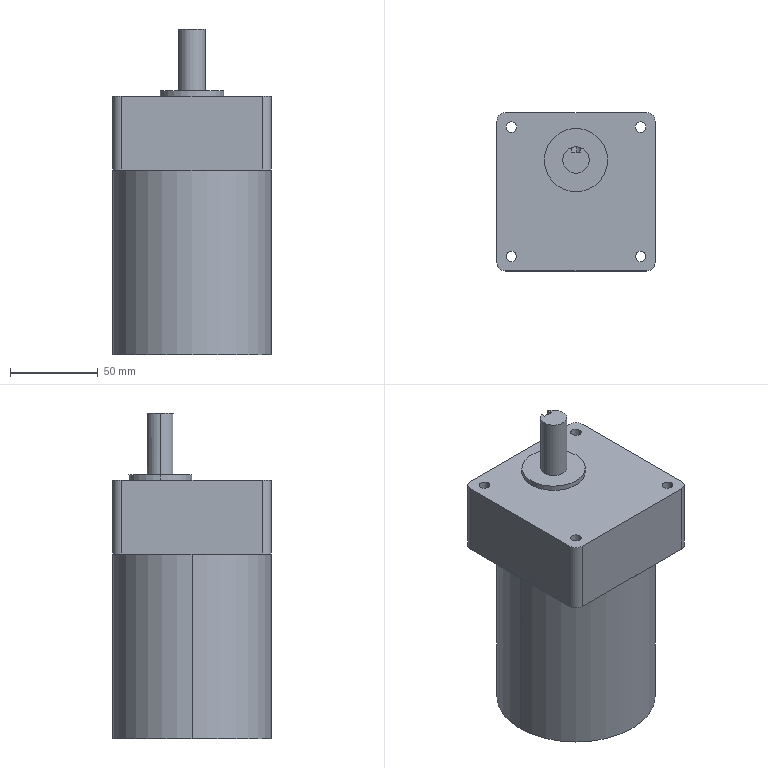Component | SolidWorks | YN90G60 90JA40G15-1 | 1 solid | 35 faces | box 90 x 90 x 185 mm | volume 1011347 mm3 | cylinder 20 | plane 15 | commonest cylinder face diameters 6 x8 10 x4 90 x2 15 x2 36 x2 5 x2
STEP:
#1=CARTESIAN_POINT('',(-1.772,4.705,-1.457));
#2=VERTEX_POINT('',#1);
#3=CARTESIAN_POINT('',(1.772,4.705,-1.457));
#4=VERTEX_POINT('',#3);
#5=CARTESIAN_POINT('',(0.,4.705,-1.457));
#6=DIRECTION('',(0.,0.,-1.));
#7=DIRECTION('',(-1.,0.,0.));
#8=AXIS2_PLACEMENT_3D('',#5,#6,#7);
#9=CIRCLE('',#8,1.772);
#10=EDGE_CURVE('',#2,#4,#9,.T.);
#11=ORIENTED_EDGE('',*,*,#10,.F.);
#12=CARTESIAN_POINT('',(-1.772,4.705,2.677));
#13=VERTEX_POINT('',#12);
#14=CARTESIAN_POINT('',(-1.772,4.705,-1.457));
#15=DIRECTION('',(0.,0.,1.));
#16=VECTOR('',#15,39.37);
#17=LINE('',#14,#16);
#18=EDGE_CURVE('',#2,#13,#17,.T.);
#19=ORIENTED_EDGE('',*,*,#18,.T.);
#20=CARTESIAN_POINT('',(0.,6.476,2.677));
#21=VERTEX_POINT('',#20);
#22=CARTESIAN_POINT('',(0.,4.705,2.677));
#23=DIRECTION('',(0.,0.,-1.));
#24=DIRECTION('',(-1.,0.,0.));
#25=AXIS2_PLACEMENT_3D('',#22,#23,#24);
#26=CIRCLE('',#25,1.772);
#27=EDGE_CURVE('',#13,#21,#26,.T.);
#28=ORIENTED_EDGE('',*,*,#27,.T.);
#29=CARTESIAN_POINT('',(1.772,4.705,2.677));
#30=VERTEX_POINT('',#29);
#31=CARTESIAN_POINT('',(0.,4.705,2.677));
#32=DIRECTION('',(0.,0.,-1.));
#33=DIRECTION('',(-1.,0.,0.));
#34=AXIS2_PLACEMENT_3D('',#31,#32,#33);
#35=CIRCLE('',#34,1.772);
#36=EDGE_CURVE('',#21,#30,#35,.T.);
#37=ORIENTED_EDGE('',*,*,#36,.T.);
#38=CARTESIAN_POINT('',(1.772,4.705,-1.457));
#39=DIRECTION('',(0.,0.,1.));
#40=VECTOR('',#39,39.37);
#41=LINE('',#38,#40);
#42=EDGE_CURVE('',#4,#30,#41,.T.);
#43=ORIENTED_EDGE('',*,*,#42,.F.);
#44=EDGE_LOOP('',(#11,#19,#28,#37,#43));
#45=FACE_OUTER_BOUND('',#44,.T.);
#46=CARTESIAN_POINT('',(0.,4.705,-1.457));
#47=DIRECTION('',(0.,0.,1.));
#48=DIRECTION('',(1.,0.,0.));
#49=AXIS2_PLACEMENT_3D('',#46,#47,#48);
#50=CYLINDRICAL_SURFACE('',#49,1.772);
#51=ADVANCED_FACE('',(#45),#50,.T.);
#52=CARTESIAN_POINT('',(0.2953,5.413,5.827));
#53=VERTEX_POINT('',#52);
#54=CARTESIAN_POINT('',(0.09843,5.692,5.827));
#55=VERTEX_POINT('',#54);
#56=CARTESIAN_POINT('',(0.,5.413,5.827));
#57=DIRECTION('',(0.,0.,1.));
#58=DIRECTION('',(1.,0.,0.));
#59=AXIS2_PLACEMENT_3D('',#56,#57,#58);
#60=CIRCLE('',#59,0.2953);
#61=EDGE_CURVE('',#53,#55,#60,.T.);
#62=ORIENTED_EDGE('',*,*,#61,.F.);
#63=CARTESIAN_POINT('',(0.2953,5.413,4.449));
#64=VERTEX_POINT('',#63);
#65=CARTESIAN_POINT('',(0.2953,5.413,5.827));
#66=DIRECTION('',(0.,0.,-1.));
#67=VECTOR('',#66,39.37);
#68=LINE('',#65,#67);
#69=EDGE_CURVE('',#53,#64,#68,.T.);
#70=ORIENTED_EDGE('',*,*,#69,.T.);
#71=CARTESIAN_POINT('',(-0.2953,5.413,4.449));
#72=VERTEX_POINT('',#71);
#73=CARTESIAN_POINT('',(0.,5.413,4.449));
#74=DIRECTION('',(0.,0.,1.));
#75=DIRECTION('',(1.,0.,0.));
#76=AXIS2_PLACEMENT_3D('',#73,#74,#75);
#77=CIRCLE('',#76,0.2953);
#78=EDGE_CURVE('',#64,#72,#77,.T.);
#79=ORIENTED_EDGE('',*,*,#78,.T.);
#80=CARTESIAN_POINT('',(-0.2953,5.413,5.827));
#81=VERTEX_POINT('',#80);
#82=CARTESIAN_POINT('',(-0.2953,5.413,5.827));
#83=DIRECTION('',(0.,0.,-1.));
#84=VECTOR('',#83,39.37);
#85=LINE('',#82,#84);
#86=EDGE_CURVE('',#81,#72,#85,.T.);
#87=ORIENTED_EDGE('',*,*,#86,.F.);
#88=CARTESIAN_POINT('',(-0.09843,5.692,5.827));
#89=VERTEX_POINT('',#88);
#90=CARTESIAN_POINT('',(0.,5.413,5.827));
#91=DIRECTION('',(0.,0.,1.));
#92=DIRECTION('',(1.,0.,0.));
#93=AXIS2_PLACEMENT_3D('',#90,#91,#92);
#94=CIRCLE('',#93,0.2953);
#95=EDGE_CURVE('',#89,#81,#94,.T.);
#96=ORIENTED_EDGE('',*,*,#95,.F.);
#97=CARTESIAN_POINT('',(-0.09843,5.692,4.744));
#98=VERTEX_POINT('',#97);
#99=CARTESIAN_POINT('',(-0.09843,5.692,5.827));
#100=DIRECTION('',(0.,0.,-1.));
#101=VECTOR('',#100,39.37);
#102=LINE('',#99,#101);
#103=EDGE_CURVE('',#89,#98,#102,.T.);
#104=ORIENTED_EDGE('',*,*,#103,.T.);
#105=CARTESIAN_POINT('',(0.,5.709,4.646));
#106=VERTEX_POINT('',#105);
#107=CARTESIAN_POINT('',(-0.09843,5.692,4.744));
#108=CARTESIAN_POINT('',(-0.09843,5.692,4.738));
#109=CARTESIAN_POINT('',(-0.09778,5.692,4.731));
#110=CARTESIAN_POINT('',(-0.09525,5.693,4.718));
#111=CARTESIAN_POINT('',(-0.09334,5.694,4.712));
#112=CARTESIAN_POINT('',(-0.08839,5.695,4.7));
#113=CARTESIAN_POINT('',(-0.08537,5.696,4.695));
#114=CARTESIAN_POINT('',(-0.07824,5.698,4.684));
#115=CARTESIAN_POINT('',(-0.07412,5.699,4.679));
#116=CARTESIAN_POINT('',(-0.06062,5.703,4.666));
#117=CARTESIAN_POINT('',(-0.04973,5.705,4.658));
#118=CARTESIAN_POINT('',(-0.032,5.707,4.651));
#119=CARTESIAN_POINT('',(-0.02576,5.708,4.649));
#120=CARTESIAN_POINT('',(-0.01301,5.708,4.646));
#121=CARTESIAN_POINT('',(-0.006549,5.709,4.646));
#122=CARTESIAN_POINT('',(0.,5.709,4.646));
#123=B_SPLINE_CURVE_WITH_KNOTS('',3,(#107,#108,#109,#110,#111,#112,#113,#114,#115,#116,#117,#118,#119,#120,#121,#122),.UNSPECIFIED.,.F.,.F.,(4,2,2,2,2,2,2,4),(0.,0.0004917,0.0009834,0.001475,0.001967,0.00295,0.003442,0.003934),.UNSPECIFIED.);
#124=EDGE_CURVE('',#98,#106,#123,.T.);
#125=ORIENTED_EDGE('',*,*,#124,.T.);
#126=CARTESIAN_POINT('',(0.09843,5.692,4.744));
#127=VERTEX_POINT('',#126);
#128=CARTESIAN_POINT('',(0.,5.709,4.646));
#129=CARTESIAN_POINT('',(0.00655,5.709,4.646));
#130=CARTESIAN_POINT('',(0.01298,5.708,4.646));
#131=CARTESIAN_POINT('',(0.02562,5.708,4.649));
#132=CARTESIAN_POINT('',(0.03189,5.707,4.651));
#133=CARTESIAN_POINT('',(0.04379,5.705,4.656));
#134=CARTESIAN_POINT('',(0.04942,5.705,4.659));
#135=CARTESIAN_POINT('',(0.06008,5.703,4.666));
#136=CARTESIAN_POINT('',(0.06509,5.701,4.67));
#137=CARTESIAN_POINT('',(0.0786,5.698,4.683));
#138=CARTESIAN_POINT('',(0.08591,5.696,4.694));
#139=CARTESIAN_POINT('',(0.0933,5.694,4.712));
#140=CARTESIAN_POINT('',(0.09522,5.693,4.718));
#141=CARTESIAN_POINT('',(0.09778,5.692,4.731));
#142=CARTESIAN_POINT('',(0.09843,5.692,4.738));
#143=CARTESIAN_POINT('',(0.09843,5.692,4.744));
#144=B_SPLINE_CURVE_WITH_KNOTS('',3,(#128,#129,#130,#131,#132,#133,#134,#135,#136,#137,#138,#139,#140,#141,#142,#143),.UNSPECIFIED.,.F.,.F.,(4,2,2,2,2,2,2,4),(0.,0.0004917,0.0009835,0.001475,0.001967,0.00295,0.003442,0.003934),.UNSPECIFIED.);
#145=EDGE_CURVE('',#106,#127,#144,.T.);
#146=ORIENTED_EDGE('',*,*,#145,.T.);
#147=CARTESIAN_POINT('',(0.09843,5.692,5.827));
#148=DIRECTION('',(0.,0.,1.));
#149=VECTOR('',#148,39.37);
#150=LINE('',#147,#149);
#151=EDGE_CURVE('',#127,#55,#150,.T.);
#152=ORIENTED_EDGE('',*,*,#151,.T.);
#153=EDGE_LOOP('',(#62,#70,#79,#87,#96,#104,#125,#146,#152));
#154=FACE_OUTER_BOUND('',#153,.T.);
#155=CARTESIAN_POINT('',(0.,5.413,5.827));
#156=DIRECTION('',(0.,0.,-1.));
#157=DIRECTION('',(-1.,0.,0.));
#158=AXIS2_PLACEMENT_3D('',#155,#156,#157);
#159=CYLINDRICAL_SURFACE('',#158,0.2953);
#160=ADVANCED_FACE('',(#154),#159,.T.);
#161=CARTESIAN_POINT('',(0.7087,5.413,4.449));
#162=VERTEX_POINT('',#161);
#163=CARTESIAN_POINT('',(-0.7087,5.413,4.449));
#164=VERTEX_POINT('',#163);
#165=CARTESIAN_POINT('',(0.,5.413,4.449));
#166=DIRECTION('',(0.,0.,1.));
#167=DIRECTION('',(1.,0.,0.));
#168=AXIS2_PLACEMENT_3D('',#165,#166,#167);
#169=CIRCLE('',#168,0.7087);
#170=EDGE_CURVE('',#162,#164,#169,.T.);
#171=ORIENTED_EDGE('',*,*,#170,.F.);
#172=CARTESIAN_POINT('',(0.7087,5.413,4.331));
#173=VERTEX_POINT('',#172);
#174=CARTESIAN_POINT('',(0.7087,5.413,4.449));
#175=DIRECTION('',(0.,0.,-1.));
#176=VECTOR('',#175,39.37);
#177=LINE('',#174,#176);
#178=EDGE_CURVE('',#162,#173,#177,.T.);
#179=ORIENTED_EDGE('',*,*,#178,.T.);
#180=CARTESIAN_POINT('',(-0.7087,5.413,4.331));
#181=VERTEX_POINT('',#180);
#182=CARTESIAN_POINT('',(0.,5.413,4.331));
#183=DIRECTION('',(0.,0.,1.));
#184=DIRECTION('',(1.,0.,0.));
#185=AXIS2_PLACEMENT_3D('',#182,#183,#184);
#186=CIRCLE('',#185,0.7087);
#187=EDGE_CURVE('',#173,#181,#186,.T.);
#188=ORIENTED_EDGE('',*,*,#187,.T.);
#189=CARTESIAN_POINT('',(-0.7087,5.413,4.449));
#190=DIRECTION('',(0.,0.,-1.));
#191=VECTOR('',#190,39.37);
#192=LINE('',#189,#191);
#193=EDGE_CURVE('',#164,#181,#192,.T.);
#194=ORIENTED_EDGE('',*,*,#193,.F.);
#195=EDGE_LOOP('',(#171,#179,#188,#194));
#196=FACE_OUTER_BOUND('',#195,.T.);
#197=CARTESIAN_POINT('',(0.,5.413,4.449));
#198=DIRECTION('',(0.,0.,-1.));
#199=DIRECTION('',(-1.,0.,0.));
#200=AXIS2_PLACEMENT_3D('',#197,#198,#199);
#201=CYLINDRICAL_SURFACE('',#200,0.7087);
#202=ADVANCED_FACE('',(#196),#201,.T.);
#203=CARTESIAN_POINT('',(1.33,3.257,4.331));
#204=VERTEX_POINT('',#203);
#205=CARTESIAN_POINT('',(1.566,3.257,4.331));
#206=VERTEX_POINT('',#205);
#207=CARTESIAN_POINT('',(1.448,3.257,4.331));
#208=DIRECTION('',(0.,0.,1.));
#209=DIRECTION('',(1.,0.,0.));
#210=AXIS2_PLACEMENT_3D('',#207,#208,#209);
#211=CIRCLE('',#210,0.1181);
#212=EDGE_CURVE('',#204,#206,#211,.T.);
#213=ORIENTED_EDGE('',*,*,#212,.T.);
#214=CARTESIAN_POINT('',(1.566,3.257,2.677));
#215=VERTEX_POINT('',#214);
#216=CARTESIAN_POINT('',(1.566,3.257,4.331));
#217=DIRECTION('',(0.,0.,-1.));
#218=VECTOR('',#217,39.37);
#219=LINE('',#216,#218);
#220=EDGE_CURVE('',#206,#215,#219,.T.);
#221=ORIENTED_EDGE('',*,*,#220,.T.);
#222=CARTESIAN_POINT('',(1.33,3.257,2.677));
#223=VERTEX_POINT('',#222);
#224=CARTESIAN_POINT('',(1.448,3.257,2.677));
#225=DIRECTION('',(0.,0.,1.));
#226=DIRECTION('',(1.,0.,0.));
#227=AXIS2_PLACEMENT_3D('',#224,#225,#226);
#228=CIRCLE('',#227,0.1181);
#229=EDGE_CURVE('',#223,#215,#228,.T.);
#230=ORIENTED_EDGE('',*,*,#229,.F.);
#231=CARTESIAN_POINT('',(1.33,3.257,4.331));
#232=DIRECTION('',(0.,0.,-1.));
#233=VECTOR('',#232,39.37);
#234=LINE('',#231,#233);
#235=EDGE_CURVE('',#204,#223,#234,.T.);
#236=ORIENTED_EDGE('',*,*,#235,.F.);
#237=EDGE_LOOP('',(#213,#221,#230,#236));
#238=FACE_OUTER_BOUND('',#237,.T.);
#239=CARTESIAN_POINT('',(1.448,3.257,4.331));
#240=DIRECTION('',(0.,0.,-1.));
#241=DIRECTION('',(-1.,0.,0.));
#242=AXIS2_PLACEMENT_3D('',#239,#240,#241);
#243=CYLINDRICAL_SURFACE('',#242,0.1181);
#244=ADVANCED_FACE('',(#238),#243,.F.);
#245=CARTESIAN_POINT('',(-1.566,3.257,4.331));
#246=VERTEX_POINT('',#245);
#247=CARTESIAN_POINT('',(-1.33,3.257,4.331));
#248=VERTEX_POINT('',#247);
#249=CARTESIAN_POINT('',(-1.448,3.257,4.331));
#250=DIRECTION('',(0.,0.,1.));
#251=DIRECTION('',(1.,0.,0.));
#252=AXIS2_PLACEMENT_3D('',#249,#250,#251);
#253=CIRCLE('',#252,0.1181);
#254=EDGE_CURVE('',#246,#248,#253,.T.);
#255=ORIENTED_EDGE('',*,*,#254,.T.);
#256=CARTESIAN_POINT('',(-1.33,3.257,2.677));
#257=VERTEX_POINT('',#256);
#258=CARTESIAN_POINT('',(-1.33,3.257,4.331));
#259=DIRECTION('',(0.,0.,-1.));
#260=VECTOR('',#259,39.37);
#261=LINE('',#258,#260);
#262=EDGE_CURVE('',#248,#257,#261,.T.);
#263=ORIENTED_EDGE('',*,*,#262,.T.);
#264=CARTESIAN_POINT('',(-1.566,3.257,2.677));
#265=VERTEX_POINT('',#264);
#266=CARTESIAN_POINT('',(-1.448,3.257,2.677));
#267=DIRECTION('',(0.,0.,1.));
#268=DIRECTION('',(1.,0.,0.));
#269=AXIS2_PLACEMENT_3D('',#266,#267,#268);
#270=CIRCLE('',#269,0.1181);
#271=EDGE_CURVE('',#265,#257,#270,.T.);
#272=ORIENTED_EDGE('',*,*,#271,.F.);
#273=CARTESIAN_POINT('',(-1.566,3.257,4.331));
#274=DIRECTION('',(0.,0.,-1.));
#275=VECTOR('',#274,39.37);
#276=LINE('',#273,#275);
#277=EDGE_CURVE('',#246,#265,#276,.T.);
#278=ORIENTED_EDGE('',*,*,#277,.F.);
#279=EDGE_LOOP('',(#255,#263,#272,#278));
#280=FACE_OUTER_BOUND('',#279,.T.);
#281=CARTESIAN_POINT('',(-1.448,3.257,4.331));
#282=DIRECTION('',(0.,0.,-1.));
#283=DIRECTION('',(-1.,0.,0.));
#284=AXIS2_PLACEMENT_3D('',#281,#282,#283);
#285=CYLINDRICAL_SURFACE('',#284,0.1181);
#286=ADVANCED_FACE('',(#280),#285,.F.);
#287=CARTESIAN_POINT('',(-1.566,6.152,4.331));
#288=VERTEX_POINT('',#287);
#289=CARTESIAN_POINT('',(-1.33,6.152,4.331));
#290=VERTEX_POINT('',#289);
#291=CARTESIAN_POINT('',(-1.448,6.152,4.331));
#292=DIRECTION('',(0.,0.,1.));
#293=DIRECTION('',(1.,0.,0.));
#294=AXIS2_PLACEMENT_3D('',#291,#292,#293);
#295=CIRCLE('',#294,0.1181);
#296=EDGE_CURVE('',#288,#290,#295,.T.);
#297=ORIENTED_EDGE('',*,*,#296,.T.);
#298=CARTESIAN_POINT('',(-1.33,6.152,2.677));
#299=VERTEX_POINT('',#298);
#300=CARTESIAN_POINT('',(-1.33,6.152,4.331));
#301=DIRECTION('',(0.,0.,-1.));
#302=VECTOR('',#301,39.37);
#303=LINE('',#300,#302);
#304=EDGE_CURVE('',#290,#299,#303,.T.);
#305=ORIENTED_EDGE('',*,*,#304,.T.);
#306=CARTESIAN_POINT('',(-1.566,6.152,2.677));
#307=VERTEX_POINT('',#306);
#308=CARTESIAN_POINT('',(-1.448,6.152,2.677));
#309=DIRECTION('',(0.,0.,1.));
#310=DIRECTION('',(1.,0.,0.));
#311=AXIS2_PLACEMENT_3D('',#308,#309,#310);
#312=CIRCLE('',#311,0.1181);
#313=EDGE_CURVE('',#307,#299,#312,.T.);
#314=ORIENTED_EDGE('',*,*,#313,.F.);
#315=CARTESIAN_POINT('',(-1.566,6.152,4.331));
#316=DIRECTION('',(0.,0.,-1.));
#317=VECTOR('',#316,39.37);
#318=LINE('',#315,#317);
#319=EDGE_CURVE('',#288,#307,#318,.T.);
#320=ORIENTED_EDGE('',*,*,#319,.F.);
#321=EDGE_LOOP('',(#297,#305,#314,#320));
#322=FACE_OUTER_BOUND('',#321,.T.);
#323=CARTESIAN_POINT('',(-1.448,6.152,4.331));
#324=DIRECTION('',(0.,0.,-1.));
#325=DIRECTION('',(-1.,0.,0.));
#326=AXIS2_PLACEMENT_3D('',#323,#324,#325);
#327=CYLINDRICAL_SURFACE('',#326,0.1181);
#328=ADVANCED_FACE('',(#322),#327,.F.);
#329=CARTESIAN_POINT('',(1.33,6.152,4.331));
#330=VERTEX_POINT('',#329);
#331=CARTESIAN_POINT('',(1.566,6.152,4.331));
#332=VERTEX_POINT('',#331);
#333=CARTESIAN_POINT('',(1.448,6.152,4.331));
#334=DIRECTION('',(0.,0.,1.));
#335=DIRECTION('',(1.,0.,0.));
#336=AXIS2_PLACEMENT_3D('',#333,#334,#335);
#337=CIRCLE('',#336,0.1181);
#338=EDGE_CURVE('',#330,#332,#337,.T.);
#339=ORIENTED_EDGE('',*,*,#338,.T.);
#340=CARTESIAN_POINT('',(1.566,6.152,2.677));
#341=VERTEX_POINT('',#340);
#342=CARTESIAN_POINT('',(1.566,6.152,4.331));
#343=DIRECTION('',(0.,0.,-1.));
#344=VECTOR('',#343,39.37);
#345=LINE('',#342,#344);
#346=EDGE_CURVE('',#332,#341,#345,.T.);
#347=ORIENTED_EDGE('',*,*,#346,.T.);
#348=CARTESIAN_POINT('',(1.33,6.152,2.677));
#349=VERTEX_POINT('',#348);
#350=CARTESIAN_POINT('',(1.448,6.152,2.677));
#351=DIRECTION('',(0.,0.,1.));
#352=DIRECTION('',(1.,0.,0.));
#353=AXIS2_PLACEMENT_3D('',#350,#351,#352);
#354=CIRCLE('',#353,0.1181);
#355=EDGE_CURVE('',#349,#341,#354,.T.);
#356=ORIENTED_EDGE('',*,*,#355,.F.);
#357=CARTESIAN_POINT('',(1.33,6.152,4.331));
#358=DIRECTION('',(0.,0.,-1.));
#359=VECTOR('',#358,39.37);
#360=LINE('',#357,#359);
#361=EDGE_CURVE('',#330,#349,#360,.T.);
#362=ORIENTED_EDGE('',*,*,#361,.F.);
#363=EDGE_LOOP('',(#339,#347,#356,#362));
#364=FACE_OUTER_BOUND('',#363,.T.);
#365=CARTESIAN_POINT('',(1.448,6.152,4.331));
#366=DIRECTION('',(0.,0.,-1.));
#367=DIRECTION('',(-1.,0.,0.));
#368=AXIS2_PLACEMENT_3D('',#365,#366,#367);
#369=CYLINDRICAL_SURFACE('',#368,0.1181);
#370=ADVANCED_FACE('',(#364),#369,.F.);
#371=ORIENTED_EDGE('',*,*,#313,.T.);
#372=CARTESIAN_POINT('',(-1.448,6.152,2.677));
#373=DIRECTION('',(0.,0.,1.));
#374=DIRECTION('',(1.,0.,0.));
#375=AXIS2_PLACEMENT_3D('',#372,#373,#374);
#376=CIRCLE('',#375,0.1181);
#377=EDGE_CURVE('',#299,#307,#376,.T.);
#378=ORIENTED_EDGE('',*,*,#377,.T.);
#379=EDGE_LOOP('',(#371,#378));
#380=FACE_BOUND('',#379,.T.);
#381=CARTESIAN_POINT('',(-1.772,6.28,2.677));
#382=VERTEX_POINT('',#381);
#383=CARTESIAN_POINT('',(-1.772,6.476,2.677));
#384=DIRECTION('',(0.,-1.,0.));
#385=VECTOR('',#384,39.37);
#386=LINE('',#383,#385);
#387=EDGE_CURVE('',#382,#13,#386,.T.);
#388=ORIENTED_EDGE('',*,*,#387,.F.);
#389=CARTESIAN_POINT('',(-1.575,6.476,2.677));
#390=VERTEX_POINT('',#389);
#391=CARTESIAN_POINT('',(-1.575,6.28,2.677));
#392=DIRECTION('',(0.,0.,-1.));
#393=DIRECTION('',(1.,0.,0.));
#394=AXIS2_PLACEMENT_3D('',#391,#392,#393);
#395=CIRCLE('',#394,0.1969);
#396=EDGE_CURVE('',#382,#390,#395,.T.);
#397=ORIENTED_EDGE('',*,*,#396,.T.);
#398=CARTESIAN_POINT('',(1.772,6.476,2.677));
#399=DIRECTION('',(-1.,0.,0.));
#400=VECTOR('',#399,39.37);
#401=LINE('',#398,#400);
#402=EDGE_CURVE('',#21,#390,#401,.T.);
#403=ORIENTED_EDGE('',*,*,#402,.F.);
#404=ORIENTED_EDGE('',*,*,#27,.F.);
#405=EDGE_LOOP('',(#388,#397,#403,#404));
#406=FACE_OUTER_BOUND('',#405,.T.);
#407=CARTESIAN_POINT('',(-449.705,63.926,2.677));
#408=DIRECTION('',(0.,0.,1.));
#409=DIRECTION('',(1.,0.,0.));
#410=AXIS2_PLACEMENT_3D('',#407,#408,#409);
#411=PLANE('',#410);
#412=ADVANCED_FACE('',(#380,#406),#411,.F.);
#413=ORIENTED_EDGE('',*,*,#355,.T.);
#414=CARTESIAN_POINT('',(1.448,6.152,2.677));
#415=DIRECTION('',(0.,0.,1.));
#416=DIRECTION('',(1.,0.,0.));
#417=AXIS2_PLACEMENT_3D('',#414,#415,#416);
#418=CIRCLE('',#417,0.1181);
#419=EDGE_CURVE('',#341,#349,#418,.T.);
#420=ORIENTED_EDGE('',*,*,#419,.T.);
#421=EDGE_LOOP('',(#413,#420));
#422=FACE_BOUND('',#421,.T.);
#423=CARTESIAN_POINT('',(1.575,6.476,2.677));
#424=VERTEX_POINT('',#423);
#425=CARTESIAN_POINT('',(1.772,6.476,2.677));
#426=DIRECTION('',(-1.,0.,0.));
#427=VECTOR('',#426,39.37);
#428=LINE('',#425,#427);
#429=EDGE_CURVE('',#424,#21,#428,.T.);
#430=ORIENTED_EDGE('',*,*,#429,.F.);
#431=CARTESIAN_POINT('',(1.772,6.28,2.677));
#432=VERTEX_POINT('',#431);
#433=CARTESIAN_POINT('',(1.575,6.28,2.677));
#434=DIRECTION('',(0.,0.,-1.));
#435=DIRECTION('',(1.,0.,0.));
#436=AXIS2_PLACEMENT_3D('',#433,#434,#435);
#437=CIRCLE('',#436,0.1969);
#438=EDGE_CURVE('',#424,#432,#437,.T.);
#439=ORIENTED_EDGE('',*,*,#438,.T.);
#440=CARTESIAN_POINT('',(1.772,2.933,2.677));
#441=DIRECTION('',(0.,1.,0.));
#442=VECTOR('',#441,39.37);
#443=LINE('',#440,#442);
#444=EDGE_CURVE('',#30,#432,#443,.T.);
#445=ORIENTED_EDGE('',*,*,#444,.F.);
#446=ORIENTED_EDGE('',*,*,#36,.F.);
#447=EDGE_LOOP('',(#430,#439,#445,#446));
#448=FACE_OUTER_BOUND('',#447,.T.);
#449=CARTESIAN_POINT('',(-449.705,63.926,2.677));
#450=DIRECTION('',(0.,0.,1.));
#451=DIRECTION('',(1.,0.,0.));
#452=AXIS2_PLACEMENT_3D('',#449,#450,#451);
#453=PLANE('',#452);
#454=ADVANCED_FACE('',(#422,#448),#453,.F.);
#455=ORIENTED_EDGE('',*,*,#229,.T.);
#456=CARTESIAN_POINT('',(1.448,3.257,2.677));
#457=DIRECTION('',(0.,0.,1.));
#458=DIRECTION('',(1.,0.,0.));
#459=AXIS2_PLACEMENT_3D('',#456,#457,#458);
#460=CIRCLE('',#459,0.1181);
#461=EDGE_CURVE('',#215,#223,#460,.T.);
#462=ORIENTED_EDGE('',*,*,#461,.T.);
#463=EDGE_LOOP('',(#455,#462));
#464=FACE_BOUND('',#463,.T.);
#465=CARTESIAN_POINT('',(1.772,3.13,2.677));
#466=VERTEX_POINT('',#465);
#467=CARTESIAN_POINT('',(1.772,2.933,2.677));
#468=DIRECTION('',(0.,1.,0.));
#469=VECTOR('',#468,39.37);
#470=LINE('',#467,#469);
#471=EDGE_CURVE('',#466,#30,#470,.T.);
#472=ORIENTED_EDGE('',*,*,#471,.F.);
#473=CARTESIAN_POINT('',(1.575,2.933,2.677));
#474=VERTEX_POINT('',#473);
#475=CARTESIAN_POINT('',(1.575,3.13,2.677));
#476=DIRECTION('',(0.,0.,-1.));
#477=DIRECTION('',(1.,0.,0.));
#478=AXIS2_PLACEMENT_3D('',#475,#476,#477);
#479=CIRCLE('',#478,0.1969);
#480=EDGE_CURVE('',#466,#474,#479,.T.);
#481=ORIENTED_EDGE('',*,*,#480,.T.);
#482=CARTESIAN_POINT('',(0.,2.933,2.677));
#483=VERTEX_POINT('',#482);
#484=CARTESIAN_POINT('',(-1.772,2.933,2.677));
#485=DIRECTION('',(1.,0.,0.));
#486=VECTOR('',#485,39.37);
#487=LINE('',#484,#486);
#488=EDGE_CURVE('',#483,#474,#487,.T.);
#489=ORIENTED_EDGE('',*,*,#488,.F.);
#490=CARTESIAN_POINT('',(0.,4.705,2.677));
#491=DIRECTION('',(0.,0.,-1.));
#492=DIRECTION('',(-1.,0.,0.));
#493=AXIS2_PLACEMENT_3D('',#490,#491,#492);
#494=CIRCLE('',#493,1.772);
#495=EDGE_CURVE('',#30,#483,#494,.T.);
#496=ORIENTED_EDGE('',*,*,#495,.F.);
#497=EDGE_LOOP('',(#472,#481,#489,#496));
#498=FACE_OUTER_BOUND('',#497,.T.);
#499=CARTESIAN_POINT('',(-449.705,63.926,2.677));
#500=DIRECTION('',(0.,0.,1.));
#501=DIRECTION('',(1.,0.,0.));
#502=AXIS2_PLACEMENT_3D('',#499,#500,#501);
#503=PLANE('',#502);
#504=ADVANCED_FACE('',(#464,#498),#503,.F.);
#505=ORIENTED_EDGE('',*,*,#271,.T.);
#506=CARTESIAN_POINT('',(-1.448,3.257,2.677));
#507=DIRECTION('',(0.,0.,1.));
#508=DIRECTION('',(1.,0.,0.));
#509=AXIS2_PLACEMENT_3D('',#506,#507,#508);
#510=CIRCLE('',#509,0.1181);
#511=EDGE_CURVE('',#257,#265,#510,.T.);
#512=ORIENTED_EDGE('',*,*,#511,.T.);
#513=EDGE_LOOP('',(#505,#512));
#514=FACE_BOUND('',#513,.T.);
#515=CARTESIAN_POINT('',(-1.575,2.933,2.677));
#516=VERTEX_POINT('',#515);
#517=CARTESIAN_POINT('',(-1.772,2.933,2.677));
#518=DIRECTION('',(1.,0.,0.));
#519=VECTOR('',#518,39.37);
#520=LINE('',#517,#519);
#521=EDGE_CURVE('',#516,#483,#520,.T.);
#522=ORIENTED_EDGE('',*,*,#521,.F.);
#523=CARTESIAN_POINT('',(-1.772,3.13,2.677));
#524=VERTEX_POINT('',#523);
#525=CARTESIAN_POINT('',(-1.575,3.13,2.677));
#526=DIRECTION('',(0.,0.,-1.));
#527=DIRECTION('',(1.,0.,0.));
#528=AXIS2_PLACEMENT_3D('',#525,#526,#527);
#529=CIRCLE('',#528,0.1969);
#530=EDGE_CURVE('',#516,#524,#529,.T.);
#531=ORIENTED_EDGE('',*,*,#530,.T.);
#532=CARTESIAN_POINT('',(-1.772,6.476,2.677));
#533=DIRECTION('',(0.,-1.,0.));
#534=VECTOR('',#533,39.37);
#535=LINE('',#532,#534);
#536=EDGE_CURVE('',#13,#524,#535,.T.);
#537=ORIENTED_EDGE('',*,*,#536,.F.);
#538=CARTESIAN_POINT('',(0.,4.705,2.677));
#539=DIRECTION('',(0.,0.,-1.));
#540=DIRECTION('',(-1.,0.,0.));
#541=AXIS2_PLACEMENT_3D('',#538,#539,#540);
#542=CIRCLE('',#541,1.772);
#543=EDGE_CURVE('',#483,#13,#542,.T.);
#544=ORIENTED_EDGE('',*,*,#543,.F.);
#545=EDGE_LOOP('',(#522,#531,#537,#544));
#546=FACE_OUTER_BOUND('',#545,.T.);
#547=CARTESIAN_POINT('',(-449.705,63.926,2.677));
#548=DIRECTION('',(0.,0.,1.));
#549=DIRECTION('',(1.,0.,0.));
#550=AXIS2_PLACEMENT_3D('',#547,#548,#549);
#551=PLANE('',#550);
#552=ADVANCED_FACE('',(#514,#546),#551,.F.);
#553=CARTESIAN_POINT('',(0.,5.413,4.449));
#554=DIRECTION('',(0.,0.,1.));
#555=DIRECTION('',(1.,0.,0.));
#556=AXIS2_PLACEMENT_3D('',#553,#554,#555);
#557=CIRCLE('',#556,0.7087);
#558=EDGE_CURVE('',#164,#162,#557,.T.);
#559=ORIENTED_EDGE('',*,*,#558,.T.);
#560=ORIENTED_EDGE('',*,*,#170,.T.);
#561=EDGE_LOOP('',(#559,#560));
#562=FACE_OUTER_BOUND('',#561,.T.);
#563=CARTESIAN_POINT('',(0.,5.413,4.449));
#564=DIRECTION('',(0.,0.,1.));
#565=DIRECTION('',(1.,0.,0.));
#566=AXIS2_PLACEMENT_3D('',#563,#564,#565);
#567=CIRCLE('',#566,0.2953);
#568=EDGE_CURVE('',#72,#64,#567,.T.);
#569=ORIENTED_EDGE('',*,*,#568,.F.);
#570=ORIENTED_EDGE('',*,*,#78,.F.);
#571=EDGE_LOOP('',(#569,#570));
#572=FACE_BOUND('',#571,.T.);
#573=CARTESIAN_POINT('',(0.,5.413,4.449));
#574=DIRECTION('',(0.,0.,1.));
#575=DIRECTION('',(1.,0.,0.));
#576=AXIS2_PLACEMENT_3D('',#573,#574,#575);
#577=PLANE('',#576);
#578=ADVANCED_FACE('',(#562,#572),#577,.T.);
#579=ORIENTED_EDGE('',*,*,#212,.F.);
#580=CARTESIAN_POINT('',(1.448,3.257,4.331));
#581=DIRECTION('',(0.,0.,1.));
#582=DIRECTION('',(1.,0.,0.));
#583=AXIS2_PLACEMENT_3D('',#580,#581,#582);
#584=CIRCLE('',#583,0.1181);
#585=EDGE_CURVE('',#206,#204,#584,.T.);
#586=ORIENTED_EDGE('',*,*,#585,.F.);
#587=EDGE_LOOP('',(#579,#586));
#588=FACE_BOUND('',#587,.T.);
#589=ORIENTED_EDGE('',*,*,#296,.F.);
#590=CARTESIAN_POINT('',(-1.448,6.152,4.331));
#591=DIRECTION('',(0.,0.,1.));
#592=DIRECTION('',(1.,0.,0.));
#593=AXIS2_PLACEMENT_3D('',#590,#591,#592);
#594=CIRCLE('',#593,0.1181);
#595=EDGE_CURVE('',#290,#288,#594,.T.);
#596=ORIENTED_EDGE('',*,*,#595,.F.);
#597=EDGE_LOOP('',(#589,#596));
#598=FACE_BOUND('',#597,.T.);
#599=CARTESIAN_POINT('',(-1.772,6.28,4.331));
#600=VERTEX_POINT('',#599);
#601=CARTESIAN_POINT('',(-1.772,3.13,4.331));
#602=VERTEX_POINT('',#601);
#603=CARTESIAN_POINT('',(-1.772,6.476,4.331));
#604=DIRECTION('',(0.,-1.,0.));
#605=VECTOR('',#604,39.37);
#606=LINE('',#603,#605);
#607=EDGE_CURVE('',#600,#602,#606,.T.);
#608=ORIENTED_EDGE('',*,*,#607,.T.);
#609=CARTESIAN_POINT('',(-1.575,2.933,4.331));
#610=VERTEX_POINT('',#609);
#611=CARTESIAN_POINT('',(-1.575,3.13,4.331));
#612=DIRECTION('',(0.,0.,1.));
#613=DIRECTION('',(1.,0.,0.));
#614=AXIS2_PLACEMENT_3D('',#611,#612,#613);
#615=CIRCLE('',#614,0.1969);
#616=EDGE_CURVE('',#602,#610,#615,.T.);
#617=ORIENTED_EDGE('',*,*,#616,.T.);
#618=CARTESIAN_POINT('',(1.575,2.933,4.331));
#619=VERTEX_POINT('',#618);
#620=CARTESIAN_POINT('',(-1.772,2.933,4.331));
#621=DIRECTION('',(1.,0.,0.));
#622=VECTOR('',#621,39.37);
#623=LINE('',#620,#622);
#624=EDGE_CURVE('',#610,#619,#623,.T.);
#625=ORIENTED_EDGE('',*,*,#624,.T.);
#626=CARTESIAN_POINT('',(1.772,3.13,4.331));
#627=VERTEX_POINT('',#626);
#628=CARTESIAN_POINT('',(1.575,3.13,4.331));
#629=DIRECTION('',(0.,0.,1.));
#630=DIRECTION('',(1.,0.,0.));
#631=AXIS2_PLACEMENT_3D('',#628,#629,#630);
#632=CIRCLE('',#631,0.1969);
#633=EDGE_CURVE('',#619,#627,#632,.T.);
#634=ORIENTED_EDGE('',*,*,#633,.T.);
#635=CARTESIAN_POINT('',(1.772,6.28,4.331));
#636=VERTEX_POINT('',#635);
#637=CARTESIAN_POINT('',(1.772,2.933,4.331));
#638=DIRECTION('',(0.,1.,0.));
#639=VECTOR('',#638,39.37);
#640=LINE('',#637,#639);
#641=EDGE_CURVE('',#627,#636,#640,.T.);
#642=ORIENTED_EDGE('',*,*,#641,.T.);
#643=CARTESIAN_POINT('',(1.575,6.476,4.331));
#644=VERTEX_POINT('',#643);
#645=CARTESIAN_POINT('',(1.575,6.28,4.331));
#646=DIRECTION('',(0.,0.,1.));
#647=DIRECTION('',(1.,0.,0.));
#648=AXIS2_PLACEMENT_3D('',#645,#646,#647);
#649=CIRCLE('',#648,0.1969);
#650=EDGE_CURVE('',#636,#644,#649,.T.);
#651=ORIENTED_EDGE('',*,*,#650,.T.);
#652=CARTESIAN_POINT('',(-1.575,6.476,4.331));
#653=VERTEX_POINT('',#652);
#654=CARTESIAN_POINT('',(1.772,6.476,4.331));
#655=DIRECTION('',(-1.,0.,0.));
#656=VECTOR('',#655,39.37);
#657=LINE('',#654,#656);
#658=EDGE_CURVE('',#644,#653,#657,.T.);
#659=ORIENTED_EDGE('',*,*,#658,.T.);
#660=CARTESIAN_POINT('',(-1.575,6.28,4.331));
#661=DIRECTION('',(0.,0.,1.));
#662=DIRECTION('',(1.,0.,0.));
#663=AXIS2_PLACEMENT_3D('',#660,#661,#662);
#664=CIRCLE('',#663,0.1969);
#665=EDGE_CURVE('',#653,#600,#664,.T.);
#666=ORIENTED_EDGE('',*,*,#665,.T.);
#667=EDGE_LOOP('',(#608,#617,#625,#634,#642,#651,#659,#666));
#668=FACE_OUTER_BOUND('',#667,.T.);
#669=ORIENTED_EDGE('',*,*,#338,.F.);
#670=CARTESIAN_POINT('',(1.448,6.152,4.331));
#671=DIRECTION('',(0.,0.,1.));
#672=DIRECTION('',(1.,0.,0.));
#673=AXIS2_PLACEMENT_3D('',#670,#671,#672);
#674=CIRCLE('',#673,0.1181);
#675=EDGE_CURVE('',#332,#330,#674,.T.);
#676=ORIENTED_EDGE('',*,*,#675,.F.);
#677=EDGE_LOOP('',(#669,#676));
#678=FACE_BOUND('',#677,.T.);
#679=ORIENTED_EDGE('',*,*,#254,.F.);
#680=CARTESIAN_POINT('',(-1.448,3.257,4.331));
#681=DIRECTION('',(0.,0.,1.));
#682=DIRECTION('',(1.,0.,0.));
#683=AXIS2_PLACEMENT_3D('',#680,#681,#682);
#684=CIRCLE('',#683,0.1181);
#685=EDGE_CURVE('',#248,#246,#684,.T.);
#686=ORIENTED_EDGE('',*,*,#685,.F.);
#687=EDGE_LOOP('',(#679,#686));
#688=FACE_BOUND('',#687,.T.);
#689=CARTESIAN_POINT('',(0.,5.413,4.331));
#690=DIRECTION('',(0.,0.,1.));
#691=DIRECTION('',(1.,0.,0.));
#692=AXIS2_PLACEMENT_3D('',#689,#690,#691);
#693=CIRCLE('',#692,0.7087);
#694=EDGE_CURVE('',#181,#173,#693,.T.);
#695=ORIENTED_EDGE('',*,*,#694,.F.);
#696=ORIENTED_EDGE('',*,*,#187,.F.);
#697=EDGE_LOOP('',(#695,#696));
#698=FACE_BOUND('',#697,.T.);
#699=CARTESIAN_POINT('',(-449.705,63.926,4.331));
#700=DIRECTION('',(0.,0.,1.));
#701=DIRECTION('',(1.,0.,0.));
#702=AXIS2_PLACEMENT_3D('',#699,#700,#701);
#703=PLANE('',#702);
#704=ADVANCED_FACE('',(#588,#598,#668,#678,#688,#698),#703,.T.);
#705=ORIENTED_EDGE('',*,*,#641,.F.);
#706=CARTESIAN_POINT('',(1.772,3.13,4.331));
#707=DIRECTION('',(0.,0.,-1.));
#708=VECTOR('',#707,39.37);
#709=LINE('',#706,#708);
#710=EDGE_CURVE('',#627,#466,#709,.T.);
#711=ORIENTED_EDGE('',*,*,#710,.T.);
#712=ORIENTED_EDGE('',*,*,#471,.T.);
#713=ORIENTED_EDGE('',*,*,#444,.T.);
#714=CARTESIAN_POINT('',(1.772,6.28,4.331));
#715=DIRECTION('',(0.,0.,1.));
#716=VECTOR('',#715,39.37);
#717=LINE('',#714,#716);
#718=EDGE_CURVE('',#432,#636,#717,.T.);
#719=ORIENTED_EDGE('',*,*,#718,.T.);
#720=EDGE_LOOP('',(#705,#711,#712,#713,#719));
#721=FACE_OUTER_BOUND('',#720,.T.);
#722=CARTESIAN_POINT('',(1.772,2.933,4.331));
#723=DIRECTION('',(-1.,0.,0.));
#724=DIRECTION('',(0.,0.,1.));
#725=AXIS2_PLACEMENT_3D('',#722,#723,#724);
#726=PLANE('',#725);
#727=ADVANCED_FACE('',(#721),#726,.F.);
#728=ORIENTED_EDGE('',*,*,#402,.T.);
#729=CARTESIAN_POINT('',(-1.575,6.476,4.331));
#730=DIRECTION('',(0.,0.,1.));
#731=VECTOR('',#730,39.37);
#732=LINE('',#729,#731);
#733=EDGE_CURVE('',#390,#653,#732,.T.);
#734=ORIENTED_EDGE('',*,*,#733,.T.);
#735=ORIENTED_EDGE('',*,*,#658,.F.);
#736=CARTESIAN_POINT('',(1.575,6.476,4.331));
#737=DIRECTION('',(0.,0.,-1.));
#738=VECTOR('',#737,39.37);
#739=LINE('',#736,#738);
#740=EDGE_CURVE('',#644,#424,#739,.T.);
#741=ORIENTED_EDGE('',*,*,#740,.T.);
#742=ORIENTED_EDGE('',*,*,#429,.T.);
#743=EDGE_LOOP('',(#728,#734,#735,#741,#742));
#744=FACE_OUTER_BOUND('',#743,.T.);
#745=CARTESIAN_POINT('',(1.772,6.476,4.331));
#746=DIRECTION('',(0.,-1.,0.));
#747=DIRECTION('',(0.,0.,-1.));
#748=AXIS2_PLACEMENT_3D('',#745,#746,#747);
#749=PLANE('',#748);
#750=ADVANCED_FACE('',(#744),#749,.F.);
#751=ORIENTED_EDGE('',*,*,#536,.T.);
#752=CARTESIAN_POINT('',(-1.772,3.13,4.331));
#753=DIRECTION('',(0.,0.,1.));
#754=VECTOR('',#753,39.37);
#755=LINE('',#752,#754);
#756=EDGE_CURVE('',#524,#602,#755,.T.);
#757=ORIENTED_EDGE('',*,*,#756,.T.);
#758=ORIENTED_EDGE('',*,*,#607,.F.);
#759=CARTESIAN_POINT('',(-1.772,6.28,4.331));
#760=DIRECTION('',(0.,0.,-1.));
#761=VECTOR('',#760,39.37);
#762=LINE('',#759,#761);
#763=EDGE_CURVE('',#600,#382,#762,.T.);
#764=ORIENTED_EDGE('',*,*,#763,.T.);
#765=ORIENTED_EDGE('',*,*,#387,.T.);
#766=EDGE_LOOP('',(#751,#757,#758,#764,#765));
#767=FACE_OUTER_BOUND('',#766,.T.);
#768=CARTESIAN_POINT('',(-1.772,6.476,4.331));
#769=DIRECTION('',(1.,0.,0.));
#770=DIRECTION('',(0.,0.,-1.));
#771=AXIS2_PLACEMENT_3D('',#768,#769,#770);
#772=PLANE('',#771);
#773=ADVANCED_FACE('',(#767),#772,.F.);
#774=ORIENTED_EDGE('',*,*,#624,.F.);
#775=CARTESIAN_POINT('',(-1.575,2.933,4.331));
#776=DIRECTION('',(0.,0.,-1.));
#777=VECTOR('',#776,39.37);
#778=LINE('',#775,#777);
#779=EDGE_CURVE('',#610,#516,#778,.T.);
#780=ORIENTED_EDGE('',*,*,#779,.T.);
#781=ORIENTED_EDGE('',*,*,#521,.T.);
#782=ORIENTED_EDGE('',*,*,#488,.T.);
#783=CARTESIAN_POINT('',(1.575,2.933,4.331));
#784=DIRECTION('',(0.,0.,1.));
#785=VECTOR('',#784,39.37);
#786=LINE('',#783,#785);
#787=EDGE_CURVE('',#474,#619,#786,.T.);
#788=ORIENTED_EDGE('',*,*,#787,.T.);
#789=EDGE_LOOP('',(#774,#780,#781,#782,#788));
#790=FACE_OUTER_BOUND('',#789,.T.);
#791=CARTESIAN_POINT('',(-1.772,2.933,4.331));
#792=DIRECTION('',(0.,1.,0.));
#793=DIRECTION('',(0.,0.,1.));
#794=AXIS2_PLACEMENT_3D('',#791,#792,#793);
#795=PLANE('',#794);
#796=ADVANCED_FACE('',(#790),#795,.F.);
#797=ORIENTED_EDGE('',*,*,#346,.F.);
#798=ORIENTED_EDGE('',*,*,#675,.T.);
#799=ORIENTED_EDGE('',*,*,#361,.T.);
#800=ORIENTED_EDGE('',*,*,#419,.F.);
#801=EDGE_LOOP('',(#797,#798,#799,#800));
#802=FACE_OUTER_BOUND('',#801,.T.);
#803=CARTESIAN_POINT('',(1.448,6.152,4.331));
#804=DIRECTION('',(0.,0.,-1.));
#805=DIRECTION('',(-1.,0.,0.));
#806=AXIS2_PLACEMENT_3D('',#803,#804,#805);
#807=CYLINDRICAL_SURFACE('',#806,0.1181);
#808=ADVANCED_FACE('',(#802),#807,.F.);
#809=ORIENTED_EDGE('',*,*,#304,.F.);
#810=ORIENTED_EDGE('',*,*,#595,.T.);
#811=ORIENTED_EDGE('',*,*,#319,.T.);
#812=ORIENTED_EDGE('',*,*,#377,.F.);
#813=EDGE_LOOP('',(#809,#810,#811,#812));
#814=FACE_OUTER_BOUND('',#813,.T.);
#815=CARTESIAN_POINT('',(-1.448,6.152,4.331));
#816=DIRECTION('',(0.,0.,-1.));
#817=DIRECTION('',(-1.,0.,0.));
#818=AXIS2_PLACEMENT_3D('',#815,#816,#817);
#819=CYLINDRICAL_SURFACE('',#818,0.1181);
#820=ADVANCED_FACE('',(#814),#819,.F.);
#821=ORIENTED_EDGE('',*,*,#262,.F.);
#822=ORIENTED_EDGE('',*,*,#685,.T.);
#823=ORIENTED_EDGE('',*,*,#277,.T.);
#824=ORIENTED_EDGE('',*,*,#511,.F.);
#825=EDGE_LOOP('',(#821,#822,#823,#824));
#826=FACE_OUTER_BOUND('',#825,.T.);
#827=CARTESIAN_POINT('',(-1.448,3.257,4.331));
#828=DIRECTION('',(0.,0.,-1.));
#829=DIRECTION('',(-1.,0.,0.));
#830=AXIS2_PLACEMENT_3D('',#827,#828,#829);
#831=CYLINDRICAL_SURFACE('',#830,0.1181);
#832=ADVANCED_FACE('',(#826),#831,.F.);
#833=ORIENTED_EDGE('',*,*,#220,.F.);
#834=ORIENTED_EDGE('',*,*,#585,.T.);
#835=ORIENTED_EDGE('',*,*,#235,.T.);
#836=ORIENTED_EDGE('',*,*,#461,.F.);
#837=EDGE_LOOP('',(#833,#834,#835,#836));
#838=FACE_OUTER_BOUND('',#837,.T.);
#839=CARTESIAN_POINT('',(1.448,3.257,4.331));
#840=DIRECTION('',(0.,0.,-1.));
#841=DIRECTION('',(-1.,0.,0.));
#842=AXIS2_PLACEMENT_3D('',#839,#840,#841);
#843=CYLINDRICAL_SURFACE('',#842,0.1181);
#844=ADVANCED_FACE('',(#838),#843,.F.);
#845=ORIENTED_EDGE('',*,*,#178,.F.);
#846=ORIENTED_EDGE('',*,*,#558,.F.);
#847=ORIENTED_EDGE('',*,*,#193,.T.);
#848=ORIENTED_EDGE('',*,*,#694,.T.);
#849=EDGE_LOOP('',(#845,#846,#847,#848));
#850=FACE_OUTER_BOUND('',#849,.T.);
#851=CARTESIAN_POINT('',(0.,5.413,4.449));
#852=DIRECTION('',(0.,0.,-1.));
#853=DIRECTION('',(-1.,0.,0.));
#854=AXIS2_PLACEMENT_3D('',#851,#852,#853);
#855=CYLINDRICAL_SURFACE('',#854,0.7087);
#856=ADVANCED_FACE('',(#850),#855,.T.);
#857=ORIENTED_EDGE('',*,*,#69,.F.);
#858=CARTESIAN_POINT('',(0.,5.413,5.827));
#859=DIRECTION('',(0.,0.,1.));
#860=DIRECTION('',(1.,0.,0.));
#861=AXIS2_PLACEMENT_3D('',#858,#859,#860);
#862=CIRCLE('',#861,0.2953);
#863=EDGE_CURVE('',#81,#53,#862,.T.);
#864=ORIENTED_EDGE('',*,*,#863,.F.);
#865=ORIENTED_EDGE('',*,*,#86,.T.);
#866=ORIENTED_EDGE('',*,*,#568,.T.);
#867=EDGE_LOOP('',(#857,#864,#865,#866));
#868=FACE_OUTER_BOUND('',#867,.T.);
#869=CARTESIAN_POINT('',(0.,5.413,5.827));
#870=DIRECTION('',(0.,0.,-1.));
#871=DIRECTION('',(-1.,0.,0.));
#872=AXIS2_PLACEMENT_3D('',#869,#870,#871);
#873=CYLINDRICAL_SURFACE('',#872,0.2953);
#874=ADVANCED_FACE('',(#868),#873,.T.);
#875=CARTESIAN_POINT('',(-0.09843,5.591,5.827));
#876=VERTEX_POINT('',#875);
#877=CARTESIAN_POINT('',(-0.09843,5.413,5.827));
#878=DIRECTION('',(0.,-1.,0.));
#879=VECTOR('',#878,39.37);
#880=LINE('',#877,#879);
#881=EDGE_CURVE('',#89,#876,#880,.T.);
#882=ORIENTED_EDGE('',*,*,#881,.F.);
#883=ORIENTED_EDGE('',*,*,#95,.T.);
#884=ORIENTED_EDGE('',*,*,#863,.T.);
#885=ORIENTED_EDGE('',*,*,#61,.T.);
#886=CARTESIAN_POINT('',(0.09843,5.591,5.827));
#887=VERTEX_POINT('',#886);
#888=CARTESIAN_POINT('',(0.09843,5.827,5.827));
#889=DIRECTION('',(0.,1.,0.));
#890=VECTOR('',#889,39.37);
#891=LINE('',#888,#890);
#892=EDGE_CURVE('',#887,#55,#891,.T.);
#893=ORIENTED_EDGE('',*,*,#892,.F.);
#894=CARTESIAN_POINT('',(0.09843,5.591,5.827));
#895=DIRECTION('',(1.,0.,0.));
#896=VECTOR('',#895,39.37);
#897=LINE('',#894,#896);
#898=EDGE_CURVE('',#876,#887,#897,.T.);
#899=ORIENTED_EDGE('',*,*,#898,.F.);
#900=EDGE_LOOP('',(#882,#883,#884,#885,#893,#899));
#901=FACE_OUTER_BOUND('',#900,.T.);
#902=CARTESIAN_POINT('',(0.,5.413,5.827));
#903=DIRECTION('',(0.,0.,1.));
#904=DIRECTION('',(1.,0.,0.));
#905=AXIS2_PLACEMENT_3D('',#902,#903,#904);
#906=PLANE('',#905);
#907=ADVANCED_FACE('',(#901),#906,.T.);
#908=ORIENTED_EDGE('',*,*,#18,.F.);
#909=CARTESIAN_POINT('',(0.,4.705,-1.457));
#910=DIRECTION('',(0.,0.,-1.));
#911=DIRECTION('',(-1.,0.,0.));
#912=AXIS2_PLACEMENT_3D('',#909,#910,#911);
#913=CIRCLE('',#912,1.772);
#914=EDGE_CURVE('',#4,#2,#913,.T.);
#915=ORIENTED_EDGE('',*,*,#914,.F.);
#916=ORIENTED_EDGE('',*,*,#42,.T.);
#917=ORIENTED_EDGE('',*,*,#495,.T.);
#918=ORIENTED_EDGE('',*,*,#543,.T.);
#919=EDGE_LOOP('',(#908,#915,#916,#917,#918));
#920=FACE_OUTER_BOUND('',#919,.T.);
#921=CARTESIAN_POINT('',(0.,4.705,-1.457));
#922=DIRECTION('',(0.,0.,1.));
#923=DIRECTION('',(1.,0.,0.));
#924=AXIS2_PLACEMENT_3D('',#921,#922,#923);
#925=CYLINDRICAL_SURFACE('',#924,1.772);
#926=ADVANCED_FACE('',(#920),#925,.T.);
#927=ORIENTED_EDGE('',*,*,#914,.T.);
#928=ORIENTED_EDGE('',*,*,#10,.T.);
#929=EDGE_LOOP('',(#927,#928));
#930=FACE_OUTER_BOUND('',#929,.T.);
#931=CARTESIAN_POINT('',(0.,4.705,-1.457));
#932=DIRECTION('',(0.,0.,-1.));
#933=DIRECTION('',(-1.,0.,0.));
#934=AXIS2_PLACEMENT_3D('',#931,#932,#933);
#935=PLANE('',#934);
#936=ADVANCED_FACE('',(#930),#935,.T.);
#937=ORIENTED_EDGE('',*,*,#616,.F.);
#938=ORIENTED_EDGE('',*,*,#756,.F.);
#939=ORIENTED_EDGE('',*,*,#530,.F.);
#940=ORIENTED_EDGE('',*,*,#779,.F.);
#941=EDGE_LOOP('',(#937,#938,#939,#940));
#942=FACE_OUTER_BOUND('',#941,.T.);
#943=CARTESIAN_POINT('',(-1.575,3.13,4.331));
#944=DIRECTION('',(0.,0.,-1.));
#945=DIRECTION('',(-1.,0.,0.));
#946=AXIS2_PLACEMENT_3D('',#943,#944,#945);
#947=CYLINDRICAL_SURFACE('',#946,0.1969);
#948=ADVANCED_FACE('',(#942),#947,.T.);
#949=ORIENTED_EDGE('',*,*,#633,.F.);
#950=ORIENTED_EDGE('',*,*,#787,.F.);
#951=ORIENTED_EDGE('',*,*,#480,.F.);
#952=ORIENTED_EDGE('',*,*,#710,.F.);
#953=EDGE_LOOP('',(#949,#950,#951,#952));
#954=FACE_OUTER_BOUND('',#953,.T.);
#955=CARTESIAN_POINT('',(1.575,3.13,4.331));
#956=DIRECTION('',(0.,0.,-1.));
#957=DIRECTION('',(-1.,0.,0.));
#958=AXIS2_PLACEMENT_3D('',#955,#956,#957);
#959=CYLINDRICAL_SURFACE('',#958,0.1969);
#960=ADVANCED_FACE('',(#954),#959,.T.);
#961=ORIENTED_EDGE('',*,*,#665,.F.);
#962=ORIENTED_EDGE('',*,*,#733,.F.);
#963=ORIENTED_EDGE('',*,*,#396,.F.);
#964=ORIENTED_EDGE('',*,*,#763,.F.);
#965=EDGE_LOOP('',(#961,#962,#963,#964));
#966=FACE_OUTER_BOUND('',#965,.T.);
#967=CARTESIAN_POINT('',(-1.575,6.28,4.331));
#968=DIRECTION('',(0.,0.,-1.));
#969=DIRECTION('',(-1.,0.,0.));
#970=AXIS2_PLACEMENT_3D('',#967,#968,#969);
#971=CYLINDRICAL_SURFACE('',#970,0.1969);
#972=ADVANCED_FACE('',(#966),#971,.T.);
#973=ORIENTED_EDGE('',*,*,#650,.F.);
#974=ORIENTED_EDGE('',*,*,#718,.F.);
#975=ORIENTED_EDGE('',*,*,#438,.F.);
#976=ORIENTED_EDGE('',*,*,#740,.F.);
#977=EDGE_LOOP('',(#973,#974,#975,#976));
#978=FACE_OUTER_BOUND('',#977,.T.);
#979=CARTESIAN_POINT('',(1.575,6.28,4.331));
#980=DIRECTION('',(0.,0.,-1.));
#981=DIRECTION('',(-1.,0.,0.));
#982=AXIS2_PLACEMENT_3D('',#979,#980,#981);
#983=CYLINDRICAL_SURFACE('',#982,0.1969);
#984=ADVANCED_FACE('',(#978),#983,.T.);
#985=CARTESIAN_POINT('',(-0.09843,5.591,4.744));
#986=VERTEX_POINT('',#985);
#987=CARTESIAN_POINT('',(-0.09843,5.591,4.646));
#988=DIRECTION('',(0.,0.,1.));
#989=VECTOR('',#988,39.37);
#990=LINE('',#987,#989);
#991=EDGE_CURVE('',#986,#876,#990,.T.);
#992=ORIENTED_EDGE('',*,*,#991,.F.);
#993=CARTESIAN_POINT('',(-0.09843,5.692,4.744));
#994=DIRECTION('',(0.,1.,0.));
#995=VECTOR('',#994,39.37);
#996=LINE('',#993,#995);
#997=EDGE_CURVE('',#986,#98,#996,.T.);
#998=ORIENTED_EDGE('',*,*,#997,.T.);
#999=ORIENTED_EDGE('',*,*,#103,.F.);
#1000=ORIENTED_EDGE('',*,*,#881,.T.);
#1001=EDGE_LOOP('',(#992,#998,#999,#1000));
#1002=FACE_OUTER_BOUND('',#1001,.T.);
#1003=CARTESIAN_POINT('',(-0.09843,5.827,4.646));
#1004=DIRECTION('',(-1.,0.,0.));
#1005=DIRECTION('',(0.,0.,1.));
#1006=AXIS2_PLACEMENT_3D('',#1003,#1004,#1005);
#1007=PLANE('',#1006);
#1008=ADVANCED_FACE('',(#1002),#1007,.F.);
#1009=ORIENTED_EDGE('',*,*,#151,.F.);
#1010=CARTESIAN_POINT('',(0.09843,5.591,4.744));
#1011=VERTEX_POINT('',#1010);
#1012=CARTESIAN_POINT('',(0.09843,5.591,4.744));
#1013=DIRECTION('',(0.,-1.,0.));
#1014=VECTOR('',#1013,39.37);
#1015=LINE('',#1012,#1014);
#1016=EDGE_CURVE('',#127,#1011,#1015,.T.);
#1017=ORIENTED_EDGE('',*,*,#1016,.T.);
#1018=CARTESIAN_POINT('',(0.09843,5.591,4.646));
#1019=DIRECTION('',(0.,0.,1.));
#1020=VECTOR('',#1019,39.37);
#1021=LINE('',#1018,#1020);
#1022=EDGE_CURVE('',#1011,#887,#1021,.T.);
#1023=ORIENTED_EDGE('',*,*,#1022,.T.);
#1024=ORIENTED_EDGE('',*,*,#892,.T.);
#1025=EDGE_LOOP('',(#1009,#1017,#1023,#1024));
#1026=FACE_OUTER_BOUND('',#1025,.T.);
#1027=CARTESIAN_POINT('',(0.09843,5.827,4.646));
#1028=DIRECTION('',(1.,0.,0.));
#1029=DIRECTION('',(0.,0.,-1.));
#1030=AXIS2_PLACEMENT_3D('',#1027,#1028,#1029);
#1031=PLANE('',#1030);
#1032=ADVANCED_FACE('',(#1026),#1031,.F.);
#1033=ORIENTED_EDGE('',*,*,#1022,.F.);
#1034=CARTESIAN_POINT('',(0.,5.591,4.646));
#1035=VERTEX_POINT('',#1034);
#1036=CARTESIAN_POINT('',(0.,5.591,4.744));
#1037=DIRECTION('',(0.,1.,0.));
#1038=DIRECTION('',(0.,0.,-1.));
#1039=AXIS2_PLACEMENT_3D('',#1036,#1037,#1038);
#1040=CIRCLE('',#1039,0.09843);
#1041=EDGE_CURVE('',#1011,#1035,#1040,.T.);
#1042=ORIENTED_EDGE('',*,*,#1041,.T.);
#1043=CARTESIAN_POINT('',(0.,5.591,4.744));
#1044=DIRECTION('',(0.,1.,0.));
#1045=DIRECTION('',(0.,0.,-1.));
#1046=AXIS2_PLACEMENT_3D('',#1043,#1044,#1045);
#1047=CIRCLE('',#1046,0.09843);
#1048=EDGE_CURVE('',#1035,#986,#1047,.T.);
#1049=ORIENTED_EDGE('',*,*,#1048,.T.);
#1050=ORIENTED_EDGE('',*,*,#991,.T.);
#1051=ORIENTED_EDGE('',*,*,#898,.T.);
#1052=EDGE_LOOP('',(#1033,#1042,#1049,#1050,#1051));
#1053=FACE_OUTER_BOUND('',#1052,.T.);
#1054=CARTESIAN_POINT('',(0.09843,5.591,4.646));
#1055=DIRECTION('',(0.,-1.,0.));
#1056=DIRECTION('',(0.,0.,-1.));
#1057=AXIS2_PLACEMENT_3D('',#1054,#1055,#1056);
#1058=PLANE('',#1057);
#1059=ADVANCED_FACE('',(#1053),#1058,.F.);
#1060=ORIENTED_EDGE('',*,*,#997,.F.);
#1061=ORIENTED_EDGE('',*,*,#1048,.F.);
#1062=CARTESIAN_POINT('',(0.,5.591,4.646));
#1063=DIRECTION('',(0.,-1.,0.));
#1064=VECTOR('',#1063,39.37);
#1065=LINE('',#1062,#1064);
#1066=EDGE_CURVE('',#106,#1035,#1065,.T.);
#1067=ORIENTED_EDGE('',*,*,#1066,.F.);
#1068=ORIENTED_EDGE('',*,*,#124,.F.);
#1069=EDGE_LOOP('',(#1060,#1061,#1067,#1068));
#1070=FACE_OUTER_BOUND('',#1069,.T.);
#1071=CARTESIAN_POINT('',(0.,63.926,4.744));
#1072=DIRECTION('',(0.,1.,0.));
#1073=DIRECTION('',(0.,0.,1.));
#1074=AXIS2_PLACEMENT_3D('',#1071,#1072,#1073);
#1075=CYLINDRICAL_SURFACE('',#1074,0.09843);
#1076=ADVANCED_FACE('',(#1070),#1075,.F.);
#1077=ORIENTED_EDGE('',*,*,#1041,.F.);
#1078=ORIENTED_EDGE('',*,*,#1016,.F.);
#1079=ORIENTED_EDGE('',*,*,#145,.F.);
#1080=ORIENTED_EDGE('',*,*,#1066,.T.);
#1081=EDGE_LOOP('',(#1077,#1078,#1079,#1080));
#1082=FACE_OUTER_BOUND('',#1081,.T.);
#1083=CARTESIAN_POINT('',(0.,63.926,4.744));
#1084=DIRECTION('',(0.,-1.,0.));
#1085=DIRECTION('',(0.,0.,-1.));
#1086=AXIS2_PLACEMENT_3D('',#1083,#1084,#1085);
#1087=CYLINDRICAL_SURFACE('',#1086,0.09843);
#1088=ADVANCED_FACE('',(#1082),#1087,.F.);
#1089=CLOSED_SHELL('',(#51,#160,#202,#244,#286,#328,#370,#412,#454,#504,#552,#578,#704,#727,#750,#773,#796,#808,#820,#832,#844,#856,#874,#907,#926,#936,#948,#960,#972,#984,#1008,#1032,#1059,#1076,#1088));
#1090=MANIFOLD_SOLID_BREP('',#1089);
#1091=CARTESIAN_POINT('',(0.,0.,0.));
#1092=DIRECTION('',(0.,0.,1.));
#1093=DIRECTION('',(1.,0.,0.));
#1094=AXIS2_PLACEMENT_3D('',#1091,#1092,#1093);
#1095=(LENGTH_UNIT()NAMED_UNIT(*)SI_UNIT($,.METRE.));
#1096=LENGTH_MEASURE_WITH_UNIT(LENGTH_MEASURE(0.0254),#1095);
#1097=DIMENSIONAL_EXPONENTS(1.,0.,0.,0.,0.,0.,0.);
#1098=(CONVERSION_BASED_UNIT('',#1096)LENGTH_UNIT()NAMED_UNIT(#1097));
#1099=UNCERTAINTY_MEASURE_WITH_UNIT(LENGTH_MEASURE(0.00001),#1098,'','');
#1100=(NAMED_UNIT(*)PLANE_ANGLE_UNIT()SI_UNIT($,.RADIAN.));
#1101=(NAMED_UNIT(*)SI_UNIT($,.STERADIAN.)SOLID_ANGLE_UNIT());
#1102=(GEOMETRIC_REPRESENTATION_CONTEXT(3)GLOBAL_UNCERTAINTY_ASSIGNED_CONTEXT((#1099))GLOBAL_UNIT_ASSIGNED_CONTEXT((#1098,#1100,#1101))REPRESENTATION_CONTEXT('',''));
#1103=ADVANCED_BREP_SHAPE_REPRESENTATION('',(#1090,#1094),#1102);
#1104=COLOUR_RGB('',0.7922,0.8196,0.9333);
#1105=FILL_AREA_STYLE_COLOUR('',#1104);
#1106=FILL_AREA_STYLE('',(#1105));
#1107=SURFACE_STYLE_FILL_AREA(#1106);
#1108=SURFACE_SIDE_STYLE('',(#1107));
#1109=SURFACE_STYLE_USAGE(.BOTH.,#1108);
#1110=PRESENTATION_STYLE_ASSIGNMENT((#1109));
#1111=STYLED_ITEM('',(#1110),#1090);
#1112=(LENGTH_UNIT()NAMED_UNIT(*)SI_UNIT($,.METRE.));
#1113=LENGTH_MEASURE_WITH_UNIT(LENGTH_MEASURE(0.0254),#1112);
#1114=DIMENSIONAL_EXPONENTS(1.,0.,0.,0.,0.,0.,0.);
#1115=(CONVERSION_BASED_UNIT('',#1113)LENGTH_UNIT()NAMED_UNIT(#1114));
#1116=UNCERTAINTY_MEASURE_WITH_UNIT(LENGTH_MEASURE(0.00001),#1115,'','');
#1117=(NAMED_UNIT(*)PLANE_ANGLE_UNIT()SI_UNIT($,.RADIAN.));
#1118=(NAMED_UNIT(*)SI_UNIT($,.STERADIAN.)SOLID_ANGLE_UNIT());
#1119=(GEOMETRIC_REPRESENTATION_CONTEXT(3)GLOBAL_UNCERTAINTY_ASSIGNED_CONTEXT((#1116))GLOBAL_UNIT_ASSIGNED_CONTEXT((#1115,#1117,#1118))REPRESENTATION_CONTEXT('',''));
#1120=MECHANICAL_DESIGN_GEOMETRIC_PRESENTATION_REPRESENTATION('',(#1111),#1119);
#1121=PRESENTATION_LAYER_ASSIGNMENT('','',(#1111));